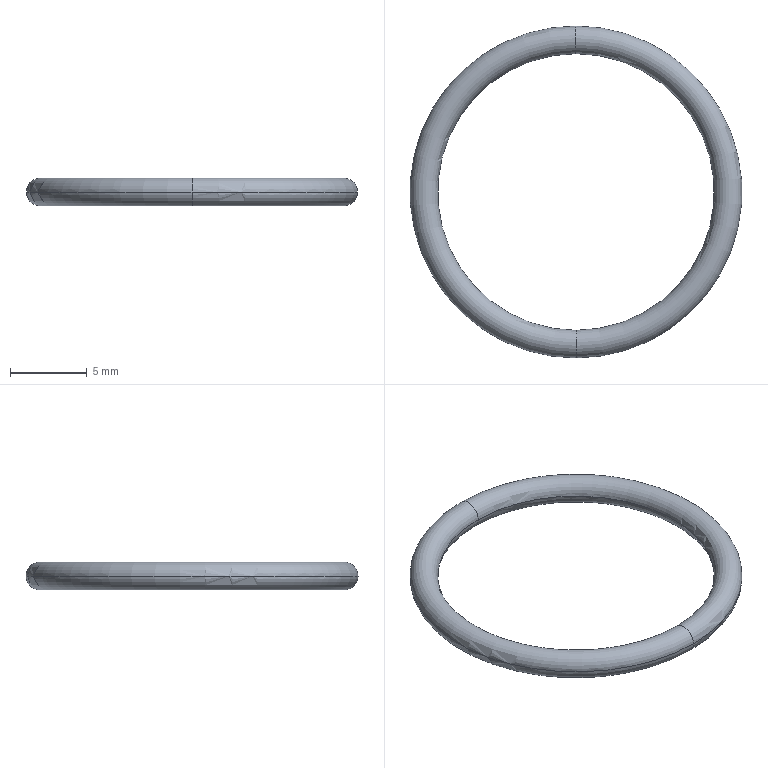Component | SolidWorks | FrontEndCapAssembly-1_GB3452.1-92O-ring18x1.8-1 | 1 solid | 4 faces | box 21.6 x 21.6 x 1.8 mm | volume 158 mm3 | torus 4
build123d program:
from build123d import *

# Parameters (mm, degrees)
SKETCH1_R = 0.9


with BuildPart() as part:
    # Sketch1 → Base-Revolve (revolve)
    with BuildSketch(Plane.XY, mode=Mode.PRIVATE) as base_revolve_sk:
        with Locations((9.9, 0)):
            Circle(SKETCH1_R)
    revolve(base_revolve_sk.sketch.rotate(Axis((0, 0, 0), (0, 1, 0)), 90), axis=Axis((0, 0, 0), (0, 1, 0)))


solid = part.part

# Placed as in the assembly
solid = solid.moved(Location((6.125, -1.646, 39.9), (90, 0, 0)))
STEP:
#1=CARTESIAN_POINT('',(0.2411,0.3604,1.571));
#2=VERTEX_POINT('',#1);
#3=CARTESIAN_POINT('',(0.2411,0.2895,1.571));
#4=VERTEX_POINT('',#3);
#5=CARTESIAN_POINT('',(0.2411,0.3249,1.571));
#6=DIRECTION('',(-1.,-0.,-0.));
#7=DIRECTION('',(0.,-1.,0.));
#8=AXIS2_PLACEMENT_3D('',#5,#6,#7);
#9=CIRCLE('',#8,0.03543);
#10=EDGE_CURVE('',#2,#4,#9,.T.);
#11=ORIENTED_EDGE('',*,*,#10,.F.);
#12=CARTESIAN_POINT('',(0.2411,-0.49,1.571));
#13=VERTEX_POINT('',#12);
#14=CARTESIAN_POINT('',(0.2411,-0.06482,1.571));
#15=DIRECTION('',(0.,0.,-1.));
#16=DIRECTION('',(-1.,0.,0.));
#17=AXIS2_PLACEMENT_3D('',#14,#15,#16);
#18=CIRCLE('',#17,0.4252);
#19=EDGE_CURVE('',#2,#13,#18,.T.);
#20=ORIENTED_EDGE('',*,*,#19,.T.);
#21=CARTESIAN_POINT('',(0.2411,-0.4192,1.571));
#22=VERTEX_POINT('',#21);
#23=CARTESIAN_POINT('',(0.2411,-0.4546,1.571));
#24=DIRECTION('',(1.,0.,0.));
#25=DIRECTION('',(-0.,1.,0.));
#26=AXIS2_PLACEMENT_3D('',#23,#24,#25);
#27=CIRCLE('',#26,0.03543);
#28=EDGE_CURVE('',#13,#22,#27,.T.);
#29=ORIENTED_EDGE('',*,*,#28,.T.);
#30=CARTESIAN_POINT('',(0.2411,-0.06482,1.571));
#31=DIRECTION('',(0.,0.,-1.));
#32=DIRECTION('',(-1.,0.,0.));
#33=AXIS2_PLACEMENT_3D('',#30,#31,#32);
#34=CIRCLE('',#33,0.3543);
#35=EDGE_CURVE('',#4,#22,#34,.T.);
#36=ORIENTED_EDGE('',*,*,#35,.F.);
#37=EDGE_LOOP('',(#11,#20,#29,#36));
#38=FACE_OUTER_BOUND('',#37,.T.);
#39=CARTESIAN_POINT('',(0.2411,-0.06482,1.571));
#40=DIRECTION('',(0.,0.,-1.));
#41=DIRECTION('',(0.,-1.,-0.));
#42=AXIS2_PLACEMENT_3D('',#39,#40,#41);
#43=TOROIDAL_SURFACE('',#42,0.3898,0.03543);
#44=ADVANCED_FACE('',(#38),#43,.T.);
#45=ORIENTED_EDGE('',*,*,#28,.F.);
#46=CARTESIAN_POINT('',(0.2411,-0.06482,1.571));
#47=DIRECTION('',(0.,0.,-1.));
#48=DIRECTION('',(-1.,0.,0.));
#49=AXIS2_PLACEMENT_3D('',#46,#47,#48);
#50=CIRCLE('',#49,0.4252);
#51=EDGE_CURVE('',#13,#2,#50,.T.);
#52=ORIENTED_EDGE('',*,*,#51,.T.);
#53=ORIENTED_EDGE('',*,*,#10,.T.);
#54=CARTESIAN_POINT('',(0.2411,-0.06482,1.571));
#55=DIRECTION('',(0.,0.,-1.));
#56=DIRECTION('',(-1.,0.,0.));
#57=AXIS2_PLACEMENT_3D('',#54,#55,#56);
#58=CIRCLE('',#57,0.3543);
#59=EDGE_CURVE('',#22,#4,#58,.T.);
#60=ORIENTED_EDGE('',*,*,#59,.F.);
#61=EDGE_LOOP('',(#45,#52,#53,#60));
#62=FACE_OUTER_BOUND('',#61,.T.);
#63=CARTESIAN_POINT('',(0.2411,-0.06482,1.571));
#64=DIRECTION('',(0.,0.,-1.));
#65=DIRECTION('',(0.,-1.,-0.));
#66=AXIS2_PLACEMENT_3D('',#63,#64,#65);
#67=TOROIDAL_SURFACE('',#66,0.3898,0.03543);
#68=ADVANCED_FACE('',(#62),#67,.T.);
#69=ORIENTED_EDGE('',*,*,#51,.F.);
#70=CARTESIAN_POINT('',(0.2411,-0.4546,1.571));
#71=DIRECTION('',(1.,0.,0.));
#72=DIRECTION('',(-0.,1.,0.));
#73=AXIS2_PLACEMENT_3D('',#70,#71,#72);
#74=CIRCLE('',#73,0.03543);
#75=EDGE_CURVE('',#22,#13,#74,.T.);
#76=ORIENTED_EDGE('',*,*,#75,.F.);
#77=ORIENTED_EDGE('',*,*,#59,.T.);
#78=CARTESIAN_POINT('',(0.2411,0.3249,1.571));
#79=DIRECTION('',(-1.,-0.,-0.));
#80=DIRECTION('',(0.,-1.,0.));
#81=AXIS2_PLACEMENT_3D('',#78,#79,#80);
#82=CIRCLE('',#81,0.03543);
#83=EDGE_CURVE('',#4,#2,#82,.T.);
#84=ORIENTED_EDGE('',*,*,#83,.T.);
#85=EDGE_LOOP('',(#69,#76,#77,#84));
#86=FACE_OUTER_BOUND('',#85,.T.);
#87=CARTESIAN_POINT('',(0.2411,-0.06482,1.571));
#88=DIRECTION('',(0.,0.,-1.));
#89=DIRECTION('',(0.,-1.,-0.));
#90=AXIS2_PLACEMENT_3D('',#87,#88,#89);
#91=TOROIDAL_SURFACE('',#90,0.3898,0.03543);
#92=ADVANCED_FACE('',(#86),#91,.T.);
#93=ORIENTED_EDGE('',*,*,#19,.F.);
#94=ORIENTED_EDGE('',*,*,#83,.F.);
#95=ORIENTED_EDGE('',*,*,#35,.T.);
#96=ORIENTED_EDGE('',*,*,#75,.T.);
#97=EDGE_LOOP('',(#93,#94,#95,#96));
#98=FACE_OUTER_BOUND('',#97,.T.);
#99=CARTESIAN_POINT('',(0.2411,-0.06482,1.571));
#100=DIRECTION('',(0.,0.,-1.));
#101=DIRECTION('',(0.,-1.,-0.));
#102=AXIS2_PLACEMENT_3D('',#99,#100,#101);
#103=TOROIDAL_SURFACE('',#102,0.3898,0.03543);
#104=ADVANCED_FACE('',(#98),#103,.T.);
#105=CLOSED_SHELL('',(#44,#68,#92,#104));
#106=MANIFOLD_SOLID_BREP('',#105);
#107=CARTESIAN_POINT('',(0.,0.,0.));
#108=DIRECTION('',(0.,0.,1.));
#109=DIRECTION('',(1.,0.,0.));
#110=AXIS2_PLACEMENT_3D('',#107,#108,#109);
#111=(LENGTH_UNIT()NAMED_UNIT(*)SI_UNIT($,.METRE.));
#112=LENGTH_MEASURE_WITH_UNIT(LENGTH_MEASURE(0.0254),#111);
#113=DIMENSIONAL_EXPONENTS(1.,0.,0.,0.,0.,0.,0.);
#114=(CONVERSION_BASED_UNIT('',#112)LENGTH_UNIT()NAMED_UNIT(#113));
#115=UNCERTAINTY_MEASURE_WITH_UNIT(LENGTH_MEASURE(0.00001),#114,'','');
#116=(NAMED_UNIT(*)PLANE_ANGLE_UNIT()SI_UNIT($,.RADIAN.));
#117=(NAMED_UNIT(*)SI_UNIT($,.STERADIAN.)SOLID_ANGLE_UNIT());
#118=(GEOMETRIC_REPRESENTATION_CONTEXT(3)GLOBAL_UNCERTAINTY_ASSIGNED_CONTEXT((#115))GLOBAL_UNIT_ASSIGNED_CONTEXT((#114,#116,#117))REPRESENTATION_CONTEXT('',''));
#119=ADVANCED_BREP_SHAPE_REPRESENTATION('',(#106,#110),#118);
#120=COLOUR_RGB('',0.7922,0.8196,0.9333);
#121=FILL_AREA_STYLE_COLOUR('',#120);
#122=FILL_AREA_STYLE('',(#121));
#123=SURFACE_STYLE_FILL_AREA(#122);
#124=SURFACE_SIDE_STYLE('',(#123));
#125=SURFACE_STYLE_USAGE(.BOTH.,#124);
#126=PRESENTATION_STYLE_ASSIGNMENT((#125));
#127=STYLED_ITEM('',(#126),#106);
#128=(LENGTH_UNIT()NAMED_UNIT(*)SI_UNIT($,.METRE.));
#129=LENGTH_MEASURE_WITH_UNIT(LENGTH_MEASURE(0.0254),#128);
#130=DIMENSIONAL_EXPONENTS(1.,0.,0.,0.,0.,0.,0.);
#131=(CONVERSION_BASED_UNIT('',#129)LENGTH_UNIT()NAMED_UNIT(#130));
#132=UNCERTAINTY_MEASURE_WITH_UNIT(LENGTH_MEASURE(0.00001),#131,'','');
#133=(NAMED_UNIT(*)PLANE_ANGLE_UNIT()SI_UNIT($,.RADIAN.));
#134=(NAMED_UNIT(*)SI_UNIT($,.STERADIAN.)SOLID_ANGLE_UNIT());
#135=(GEOMETRIC_REPRESENTATION_CONTEXT(3)GLOBAL_UNCERTAINTY_ASSIGNED_CONTEXT((#132))GLOBAL_UNIT_ASSIGNED_CONTEXT((#131,#133,#134))REPRESENTATION_CONTEXT('',''));
#136=MECHANICAL_DESIGN_GEOMETRIC_PRESENTATION_REPRESENTATION('',(#127),#135);
#137=PRESENTATION_LAYER_ASSIGNMENT('','',(#127));